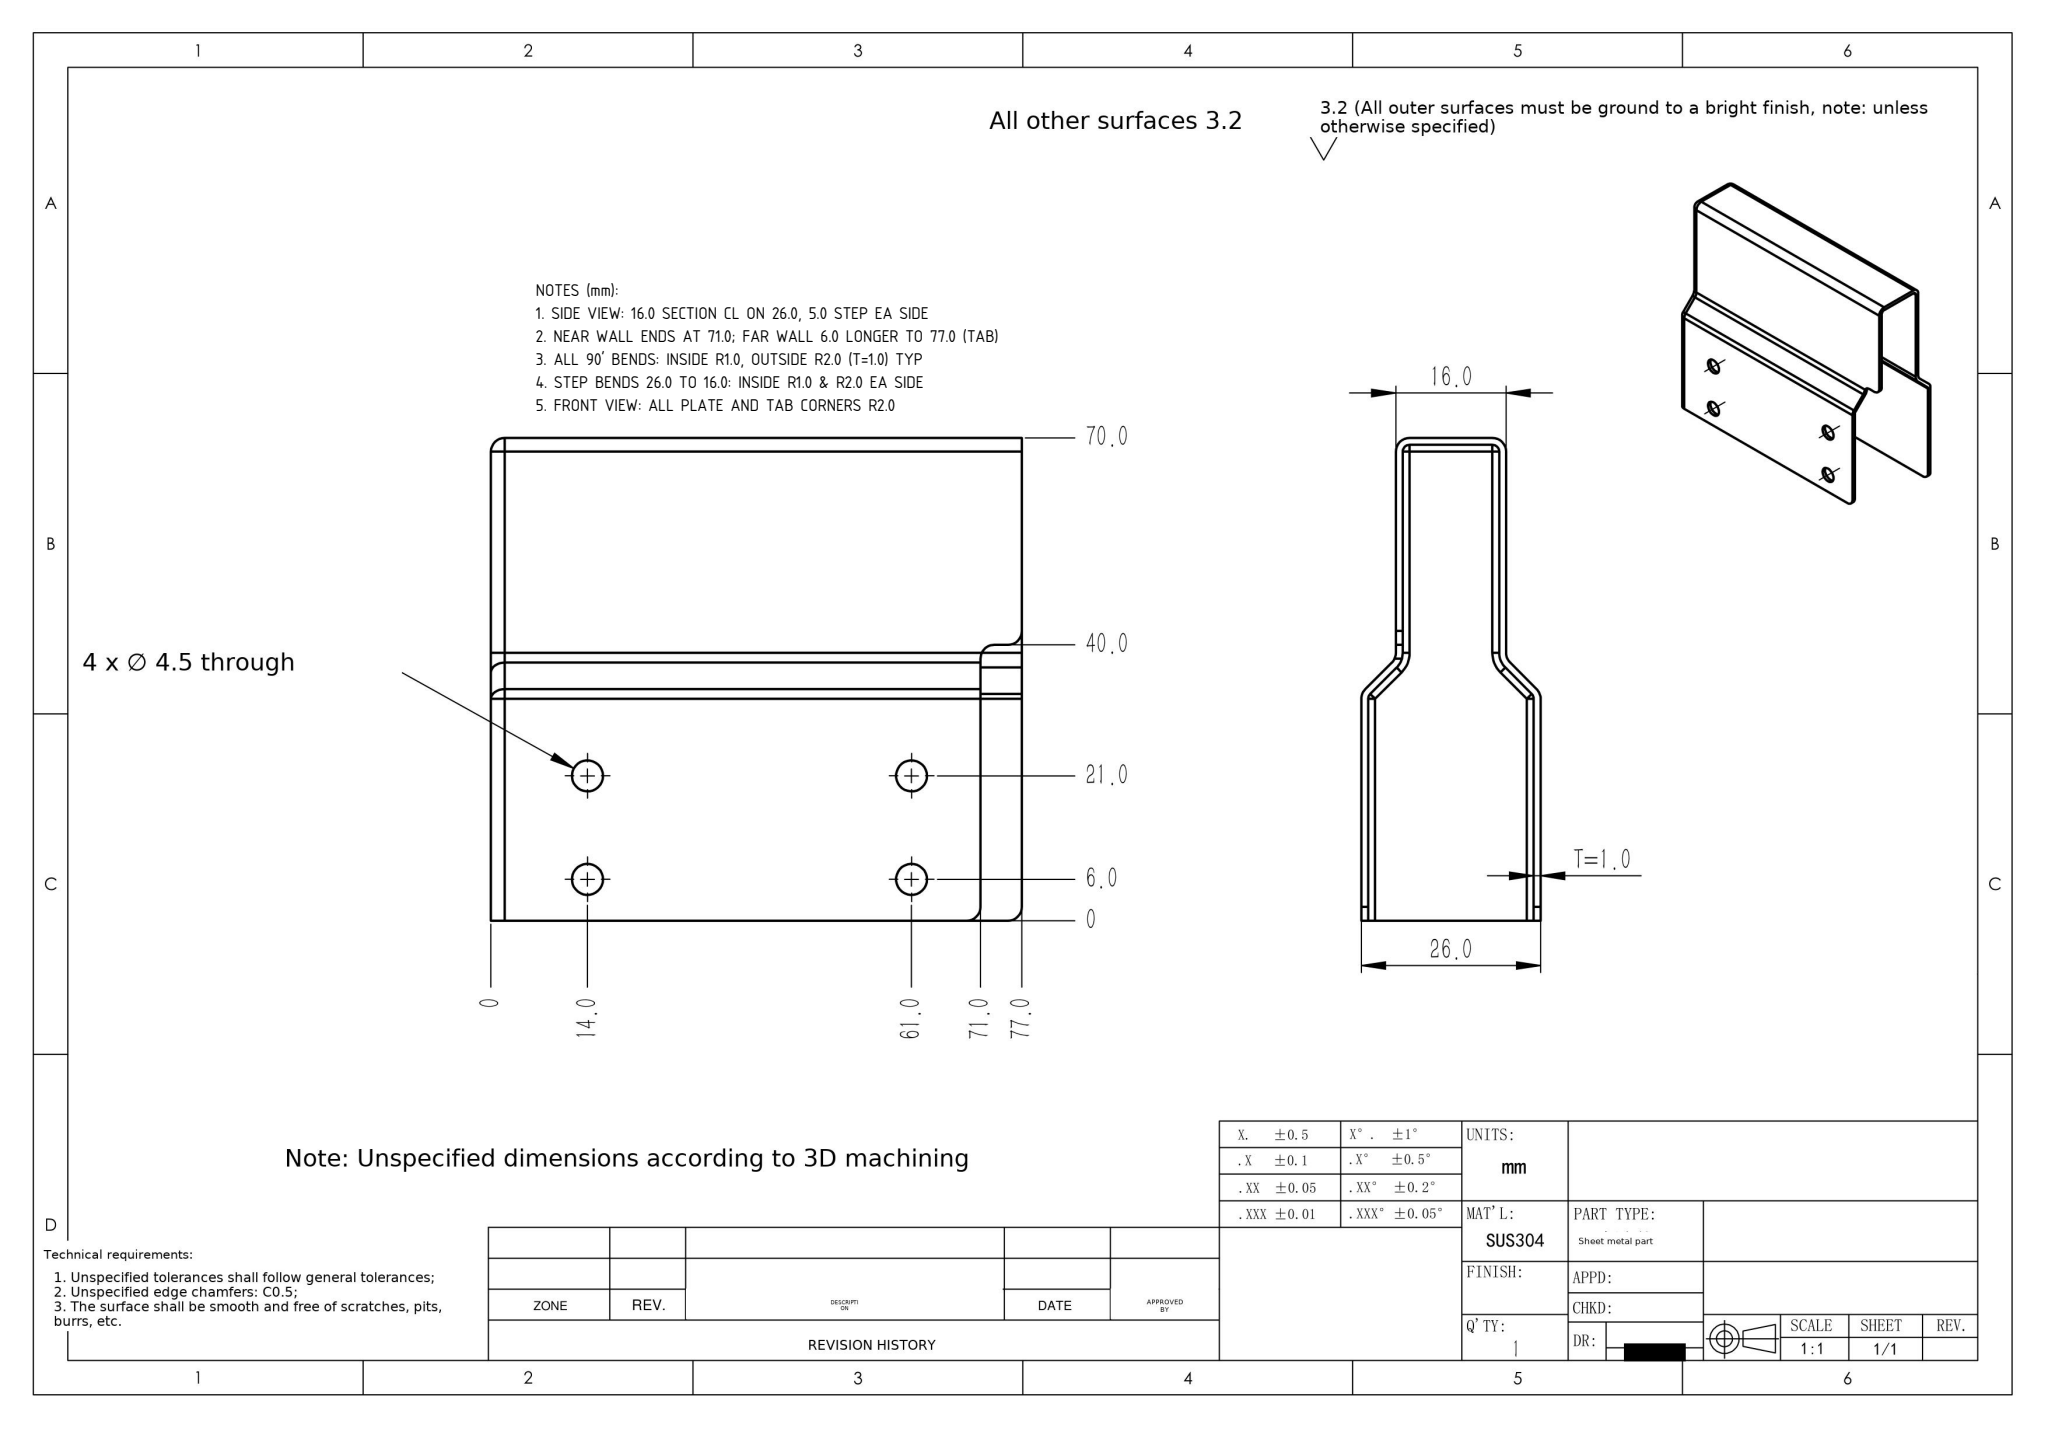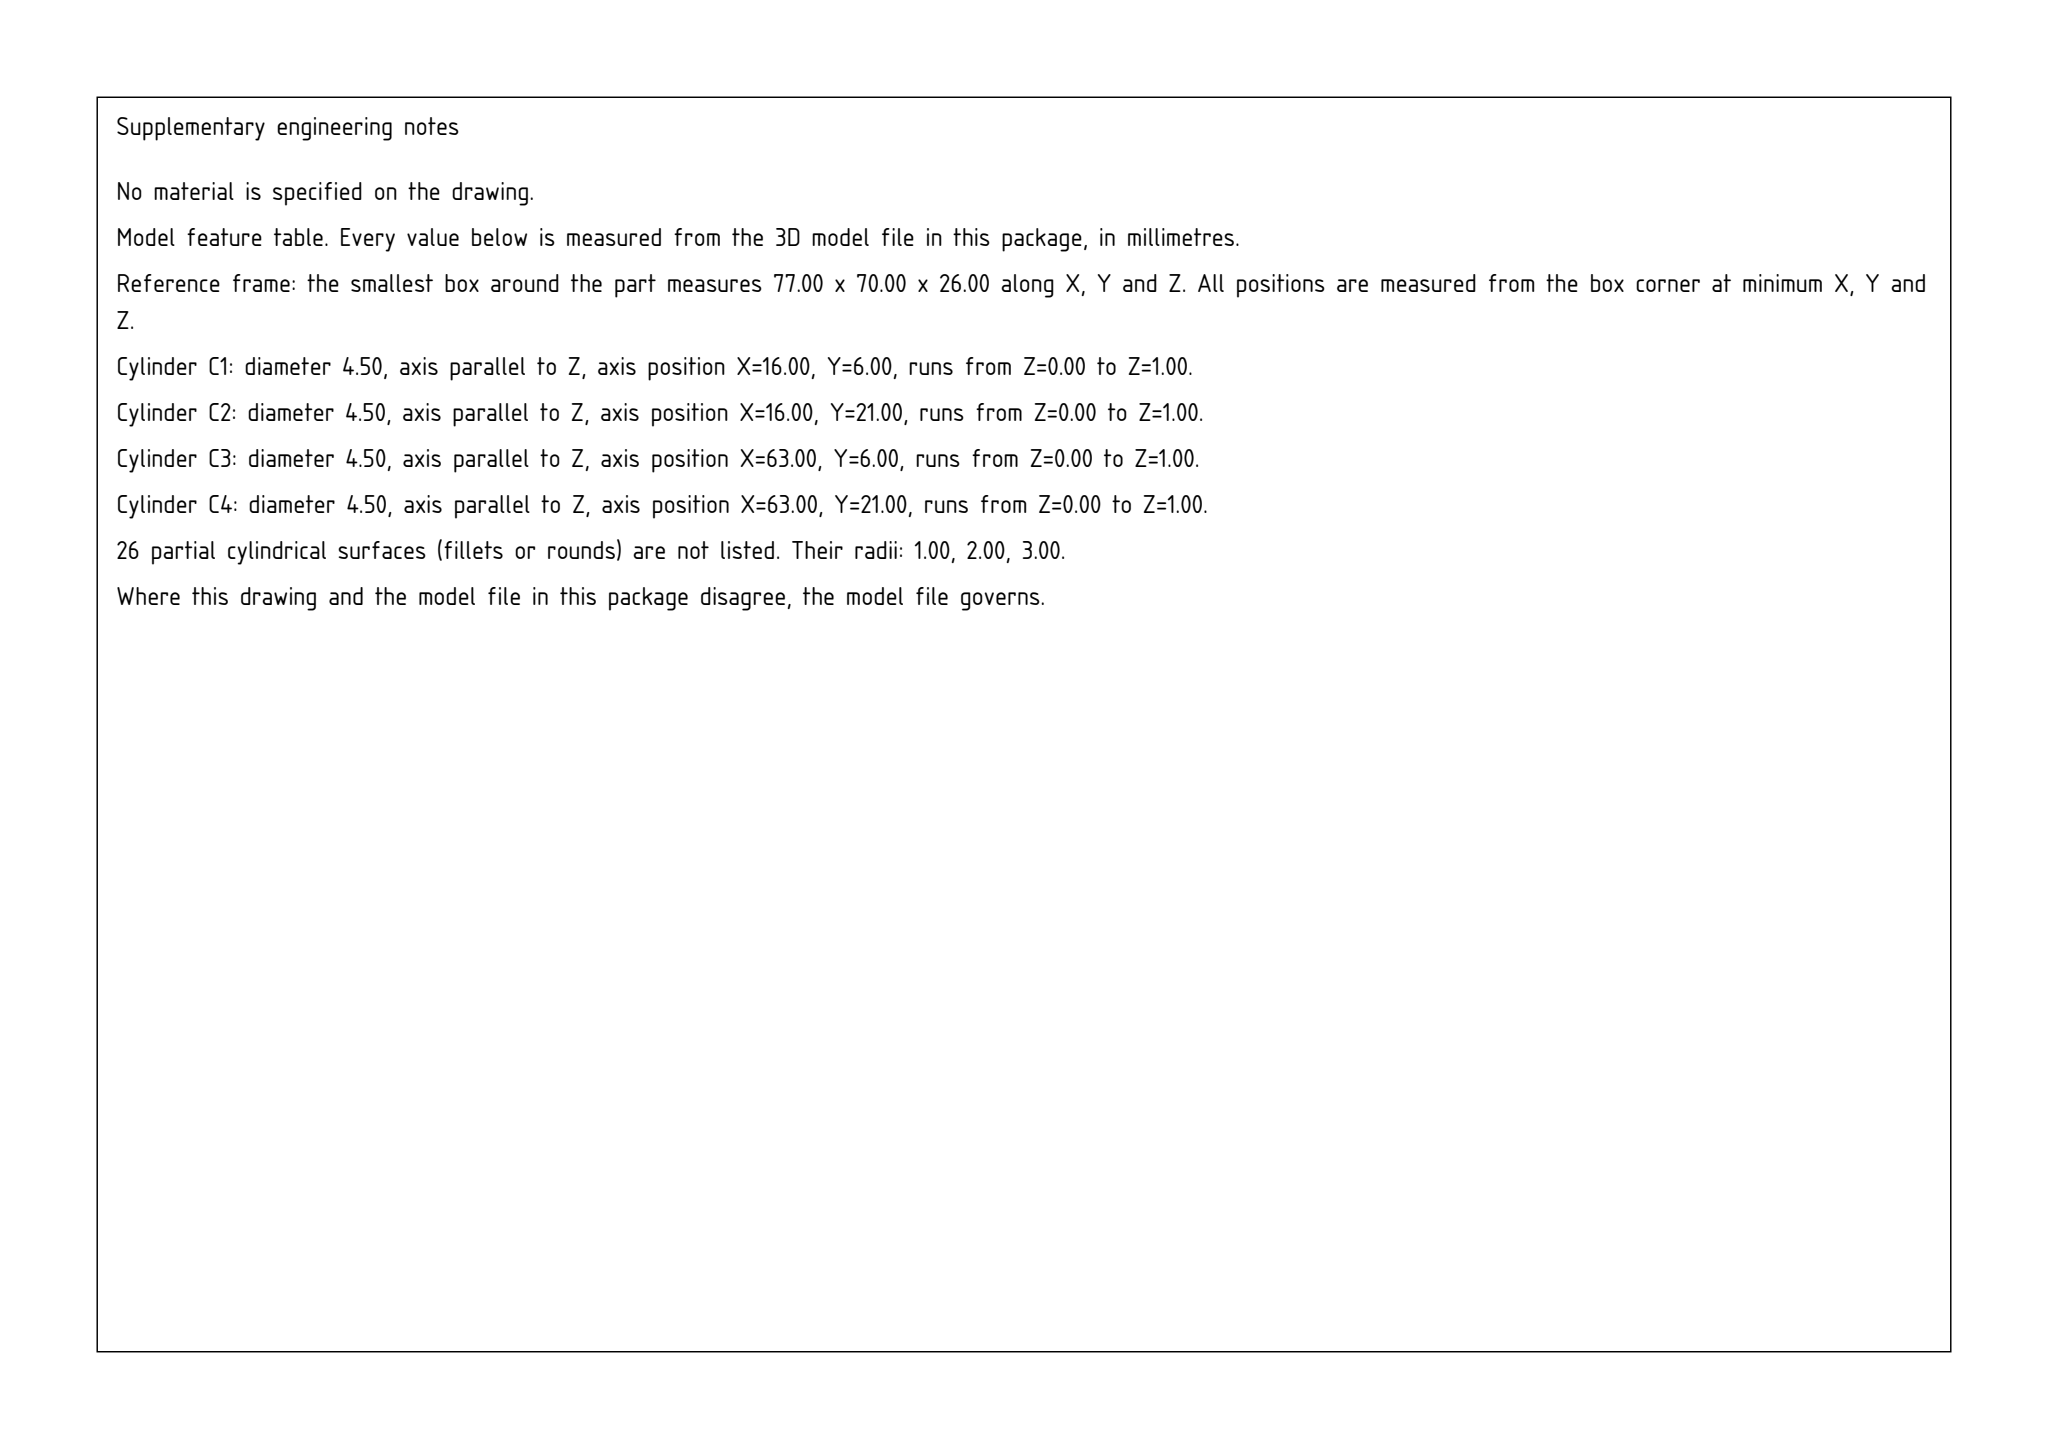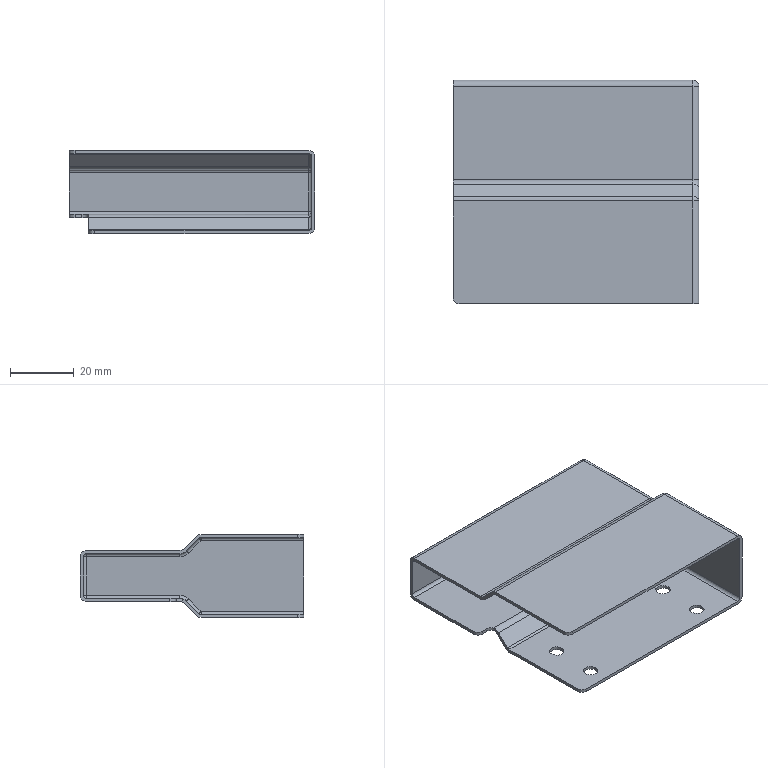Part | SolidWorks | mm | 1 solid | 70 faces | box 77 x 70 x 26 mm | volume 12950 mm3 | cylinder 38 | plane 20 | sphere 8 | torus 4 | commonest cylinder face diameters 4 x17 2 x11 4.5 x8 6 x2
Drawing notes:
SIDE VIEW: 16.0 SECTION CL ON 26.0, 5.0 STEP EA SIDE | from the solid: z-planes 0/26 (lower outer, 26 wide) and 5/21 (upper outer, 16 wide) => 5.0 step each side, symmetric
NEAR WALL ENDS AT 71.0; FAR WALL 6.0 LONGER TO 77.0 (TAB) | from the solid: x-planes at 0 and 6; bend axis x at z=2 len 69 (x 6-75) vs z=24 len 75 (x 0-75); tab at z 25-26
ALL 90' BENDS: INSIDE R1.0, OUTSIDE R2.0 (T=1.0) TYP | from the solid: Cyl dia 2.0 axis x at (y68.0,z7.0) & (y68.0,z19.0) with concentric dia 4.0 outer; fillet_radii 1.0/2.0
STEP BENDS 26.0 TO 16.0: INSIDE R1.0 & R2.0 EA SIDE | from the solid: Cyl dia 2.0/4.0 axis x at (y32.17,z2.0)&(z24.0) = R1.0 ID; cyl dia 4.0/6.0 at (y38.83,z3.0)&(z23.0) = R2.0 ID
FRONT VIEW: ALL PLATE AND TAB CORNERS R2.0 | from the solid: Cyl dia 4.0 axis z at (2.0,2.0), (8.0,2.0), (2.0,42.0), (75.0,68.0); fillet_radii 2.0